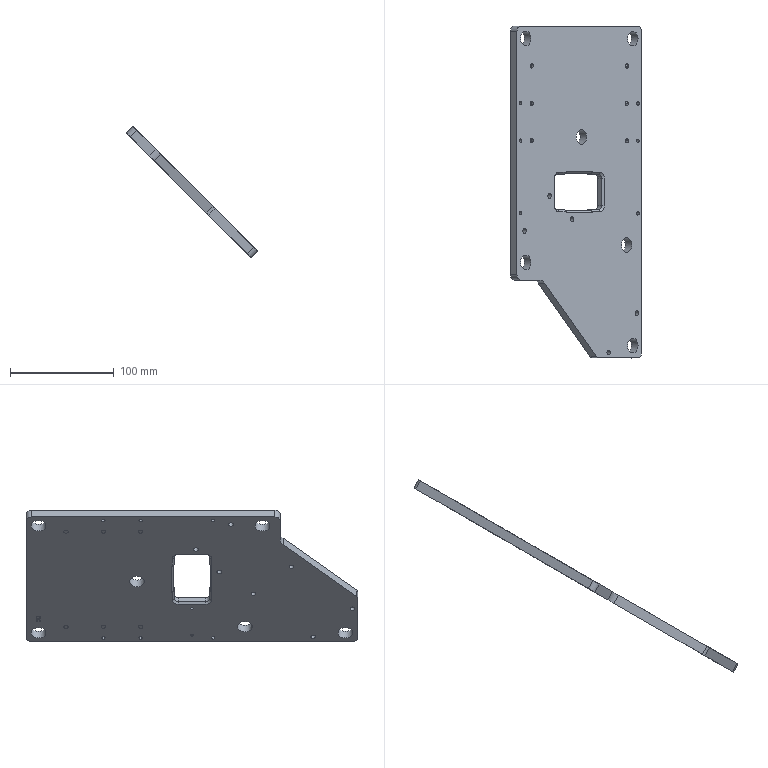CAM job | Mastercam | mm | 2 operations | part box 126.57 x 320 x 126.57
1. Contour (2D chamfer) | 7 - 6 倒角刀
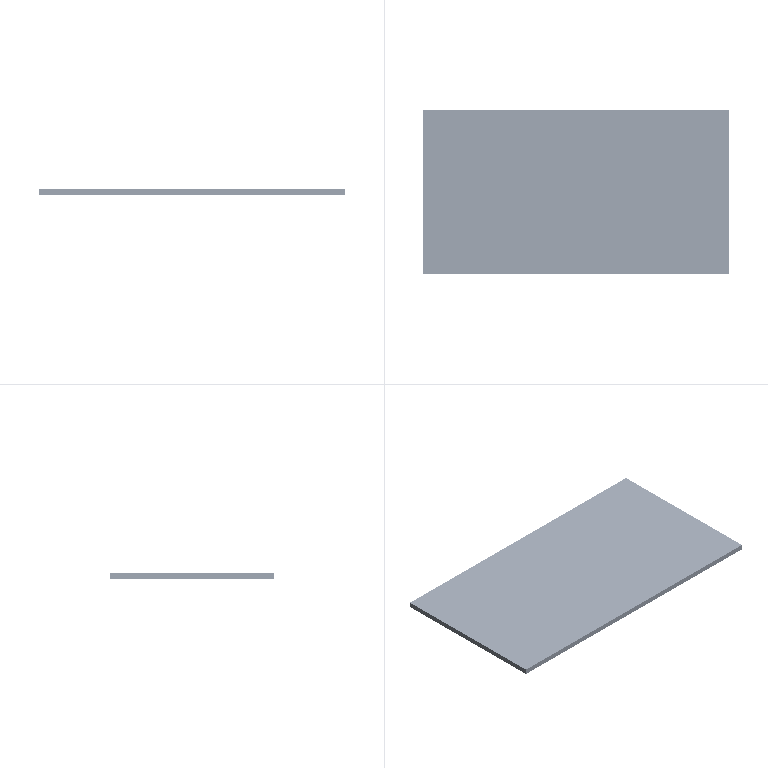2. Contour (2D chamfer) | 7 - 6 倒角刀